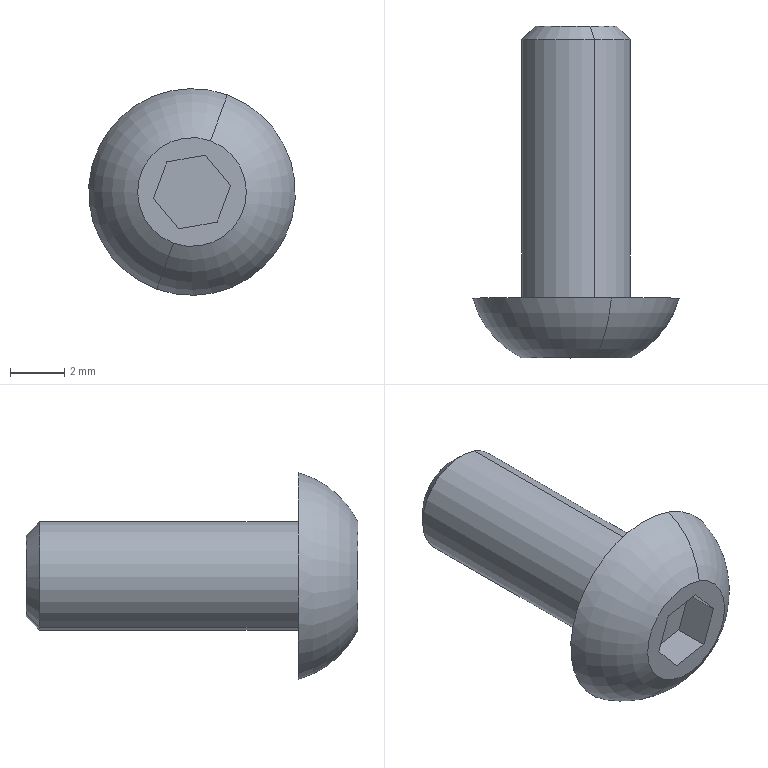Component | SolidWorks | SocketFlatHeadCapScrewM4_10-2 | 1 solid | 16 faces | box 7.6 x 12.2 x 7.6 mm | volume 188 mm3 | plane 10 | cone 2 | cylinder 2 | torus 2 | commonest cylinder face diameters 4 x2
STEP:
#1=CARTESIAN_POINT('',(-0.02018,0.5787,-2.238));
#2=VERTEX_POINT('',#1);
#3=CARTESIAN_POINT('',(0.02018,0.5787,-2.127));
#4=VERTEX_POINT('',#3);
#5=CARTESIAN_POINT('',(-0.,0.5787,-2.183));
#6=DIRECTION('',(0.,1.,0.));
#7=DIRECTION('',(-0.3417,0.,-0.9398));
#8=AXIS2_PLACEMENT_3D('',#5,#6,#7);
#9=CIRCLE('',#8,0.05906);
#10=EDGE_CURVE('',#2,#4,#9,.T.);
#11=ORIENTED_EDGE('',*,*,#10,.F.);
#12=CARTESIAN_POINT('',(-0.02691,0.5591,-2.257));
#13=VERTEX_POINT('',#12);
#14=CARTESIAN_POINT('',(-0.02018,0.5787,-2.238));
#15=DIRECTION('',(-0.2416,-0.7071,-0.6645));
#16=VECTOR('',#15,39.37);
#17=LINE('',#14,#16);
#18=EDGE_CURVE('',#2,#13,#17,.T.);
#19=ORIENTED_EDGE('',*,*,#18,.T.);
#20=CARTESIAN_POINT('',(0.02691,0.5591,-2.109));
#21=VERTEX_POINT('',#20);
#22=CARTESIAN_POINT('',(-0.,0.5591,-2.183));
#23=DIRECTION('',(-0.,-1.,-0.));
#24=DIRECTION('',(-0.3417,0.,-0.9398));
#25=AXIS2_PLACEMENT_3D('',#22,#23,#24);
#26=CIRCLE('',#25,0.07874);
#27=EDGE_CURVE('',#21,#13,#26,.T.);
#28=ORIENTED_EDGE('',*,*,#27,.F.);
#29=CARTESIAN_POINT('',(0.02018,0.5787,-2.127));
#30=DIRECTION('',(0.2416,-0.7071,0.6645));
#31=VECTOR('',#30,39.37);
#32=LINE('',#29,#31);
#33=EDGE_CURVE('',#4,#21,#32,.T.);
#34=ORIENTED_EDGE('',*,*,#33,.F.);
#35=EDGE_LOOP('',(#11,#19,#28,#34));
#36=FACE_OUTER_BOUND('',#35,.T.);
#37=CARTESIAN_POINT('',(-0.,0.5787,-2.183));
#38=DIRECTION('',(-0.,-1.,-0.));
#39=DIRECTION('',(0.3417,0.,0.9398));
#40=AXIS2_PLACEMENT_3D('',#37,#38,#39);
#41=CONICAL_SURFACE('',#40,0.05906,0.7854);
#42=ADVANCED_FACE('',(#36),#41,.T.);
#43=CARTESIAN_POINT('',(-0.02691,0.185,-2.257));
#44=VERTEX_POINT('',#43);
#45=CARTESIAN_POINT('',(0.02691,0.185,-2.109));
#46=VERTEX_POINT('',#45);
#47=CARTESIAN_POINT('',(-0.,0.185,-2.183));
#48=DIRECTION('',(0.,1.,0.));
#49=DIRECTION('',(-0.3417,0.,-0.9398));
#50=AXIS2_PLACEMENT_3D('',#47,#48,#49);
#51=CIRCLE('',#50,0.07874);
#52=EDGE_CURVE('',#44,#46,#51,.T.);
#53=ORIENTED_EDGE('',*,*,#52,.T.);
#54=CARTESIAN_POINT('',(0.02691,0.09843,-2.109));
#55=DIRECTION('',(0.,1.,0.));
#56=VECTOR('',#55,39.37);
#57=LINE('',#54,#56);
#58=EDGE_CURVE('',#46,#21,#57,.T.);
#59=ORIENTED_EDGE('',*,*,#58,.T.);
#60=ORIENTED_EDGE('',*,*,#27,.T.);
#61=CARTESIAN_POINT('',(-0.02691,0.09843,-2.257));
#62=DIRECTION('',(0.,1.,0.));
#63=VECTOR('',#62,39.37);
#64=LINE('',#61,#63);
#65=EDGE_CURVE('',#44,#13,#64,.T.);
#66=ORIENTED_EDGE('',*,*,#65,.F.);
#67=EDGE_LOOP('',(#53,#59,#60,#66));
#68=FACE_OUTER_BOUND('',#67,.T.);
#69=CARTESIAN_POINT('',(-0.,0.09843,-2.183));
#70=DIRECTION('',(0.,1.,0.));
#71=DIRECTION('',(-0.3417,0.,-0.9398));
#72=AXIS2_PLACEMENT_3D('',#69,#70,#71);
#73=CYLINDRICAL_SURFACE('',#72,0.07874);
#74=ADVANCED_FACE('',(#68),#73,.T.);
#75=CARTESIAN_POINT('',(-0.02691,0.09843,-2.257));
#76=VERTEX_POINT('',#75);
#77=CARTESIAN_POINT('',(0.02691,0.09843,-2.109));
#78=VERTEX_POINT('',#77);
#79=CARTESIAN_POINT('',(-0.,0.09843,-2.183));
#80=DIRECTION('',(0.,1.,0.));
#81=DIRECTION('',(-0.3417,0.,-0.9398));
#82=AXIS2_PLACEMENT_3D('',#79,#80,#81);
#83=CIRCLE('',#82,0.07874);
#84=EDGE_CURVE('',#76,#78,#83,.T.);
#85=ORIENTED_EDGE('',*,*,#84,.T.);
#86=CARTESIAN_POINT('',(0.05113,0.185,-2.042));
#87=VERTEX_POINT('',#86);
#88=CARTESIAN_POINT('',(0.005712,0.2215,-2.167));
#89=DIRECTION('',(-0.9398,0.,0.3417));
#90=DIRECTION('',(0.3417,0.,0.9398));
#91=AXIS2_PLACEMENT_3D('',#88,#89,#90);
#92=CIRCLE('',#91,0.1378);
#93=EDGE_CURVE('',#78,#87,#92,.T.);
#94=ORIENTED_EDGE('',*,*,#93,.T.);
#95=CARTESIAN_POINT('',(-0.05113,0.185,-2.324));
#96=VERTEX_POINT('',#95);
#97=CARTESIAN_POINT('',(-0.,0.185,-2.183));
#98=DIRECTION('',(0.,1.,0.));
#99=DIRECTION('',(-0.3417,0.,-0.9398));
#100=AXIS2_PLACEMENT_3D('',#97,#98,#99);
#101=CIRCLE('',#100,0.1496);
#102=EDGE_CURVE('',#96,#87,#101,.T.);
#103=ORIENTED_EDGE('',*,*,#102,.F.);
#104=CARTESIAN_POINT('',(-0.005712,0.2215,-2.199));
#105=DIRECTION('',(0.9398,-0.,-0.3417));
#106=DIRECTION('',(-0.3417,0.,-0.9398));
#107=AXIS2_PLACEMENT_3D('',#104,#105,#106);
#108=CIRCLE('',#107,0.1378);
#109=EDGE_CURVE('',#76,#96,#108,.T.);
#110=ORIENTED_EDGE('',*,*,#109,.F.);
#111=EDGE_LOOP('',(#85,#94,#103,#110));
#112=FACE_OUTER_BOUND('',#111,.T.);
#113=CARTESIAN_POINT('',(-0.,0.2215,-2.183));
#114=DIRECTION('',(0.,1.,0.));
#115=DIRECTION('',(-0.3417,0.,-0.9398));
#116=AXIS2_PLACEMENT_3D('',#113,#114,#115);
#117=TOROIDAL_SURFACE('',#116,0.01671,0.1378);
#118=ADVANCED_FACE('',(#112),#117,.T.);
#119=CARTESIAN_POINT('',(0.05596,0.09843,-2.173));
#120=VERTEX_POINT('',#119);
#121=CARTESIAN_POINT('',(0.01942,0.09843,-2.13));
#122=VERTEX_POINT('',#121);
#123=CARTESIAN_POINT('',(0.05596,0.09843,-2.173));
#124=DIRECTION('',(-0.643,0.,0.7658));
#125=VECTOR('',#124,39.37);
#126=LINE('',#123,#125);
#127=EDGE_CURVE('',#120,#122,#126,.T.);
#128=ORIENTED_EDGE('',*,*,#127,.F.);
#129=CARTESIAN_POINT('',(0.03654,0.09843,-2.226));
#130=VERTEX_POINT('',#129);
#131=CARTESIAN_POINT('',(0.03654,0.09843,-2.226));
#132=DIRECTION('',(0.3417,-0.,0.9398));
#133=VECTOR('',#132,39.37);
#134=LINE('',#131,#133);
#135=EDGE_CURVE('',#130,#120,#134,.T.);
#136=ORIENTED_EDGE('',*,*,#135,.F.);
#137=CARTESIAN_POINT('',(-0.01942,0.09843,-2.236));
#138=VERTEX_POINT('',#137);
#139=CARTESIAN_POINT('',(-0.01942,0.09843,-2.236));
#140=DIRECTION('',(0.9848,-0.,0.174));
#141=VECTOR('',#140,39.37);
#142=LINE('',#139,#141);
#143=EDGE_CURVE('',#138,#130,#142,.T.);
#144=ORIENTED_EDGE('',*,*,#143,.F.);
#145=CARTESIAN_POINT('',(-0.05596,0.09843,-2.193));
#146=VERTEX_POINT('',#145);
#147=CARTESIAN_POINT('',(-0.05596,0.09843,-2.193));
#148=DIRECTION('',(0.643,-0.,-0.7658));
#149=VECTOR('',#148,39.37);
#150=LINE('',#147,#149);
#151=EDGE_CURVE('',#146,#138,#150,.T.);
#152=ORIENTED_EDGE('',*,*,#151,.F.);
#153=CARTESIAN_POINT('',(-0.03654,0.09843,-2.139));
#154=VERTEX_POINT('',#153);
#155=CARTESIAN_POINT('',(-0.03654,0.09843,-2.139));
#156=DIRECTION('',(-0.3417,0.,-0.9398));
#157=VECTOR('',#156,39.37);
#158=LINE('',#155,#157);
#159=EDGE_CURVE('',#154,#146,#158,.T.);
#160=ORIENTED_EDGE('',*,*,#159,.F.);
#161=CARTESIAN_POINT('',(0.01942,0.09843,-2.13));
#162=DIRECTION('',(-0.9848,0.,-0.174));
#163=VECTOR('',#162,39.37);
#164=LINE('',#161,#163);
#165=EDGE_CURVE('',#122,#154,#164,.T.);
#166=ORIENTED_EDGE('',*,*,#165,.F.);
#167=EDGE_LOOP('',(#128,#136,#144,#152,#160,#166));
#168=FACE_BOUND('',#167,.T.);
#169=ORIENTED_EDGE('',*,*,#84,.F.);
#170=CARTESIAN_POINT('',(-0.,0.09843,-2.183));
#171=DIRECTION('',(0.,1.,0.));
#172=DIRECTION('',(-0.3417,0.,-0.9398));
#173=AXIS2_PLACEMENT_3D('',#170,#171,#172);
#174=CIRCLE('',#173,0.07874);
#175=EDGE_CURVE('',#78,#76,#174,.T.);
#176=ORIENTED_EDGE('',*,*,#175,.F.);
#177=EDGE_LOOP('',(#169,#176));
#178=FACE_OUTER_BOUND('',#177,.T.);
#179=CARTESIAN_POINT('',(-0.,0.09843,-2.183));
#180=DIRECTION('',(-0.,-1.,-0.));
#181=DIRECTION('',(0.3417,-0.,0.9398));
#182=AXIS2_PLACEMENT_3D('',#179,#180,#181);
#183=PLANE('',#182);
#184=ADVANCED_FACE('',(#168,#178),#183,.T.);
#185=ORIENTED_EDGE('',*,*,#93,.F.);
#186=ORIENTED_EDGE('',*,*,#175,.T.);
#187=ORIENTED_EDGE('',*,*,#109,.T.);
#188=CARTESIAN_POINT('',(-0.,0.185,-2.183));
#189=DIRECTION('',(0.,1.,0.));
#190=DIRECTION('',(-0.3417,0.,-0.9398));
#191=AXIS2_PLACEMENT_3D('',#188,#189,#190);
#192=CIRCLE('',#191,0.1496);
#193=EDGE_CURVE('',#87,#96,#192,.T.);
#194=ORIENTED_EDGE('',*,*,#193,.F.);
#195=EDGE_LOOP('',(#185,#186,#187,#194));
#196=FACE_OUTER_BOUND('',#195,.T.);
#197=CARTESIAN_POINT('',(-0.,0.2215,-2.183));
#198=DIRECTION('',(0.,1.,0.));
#199=DIRECTION('',(-0.3417,0.,-0.9398));
#200=AXIS2_PLACEMENT_3D('',#197,#198,#199);
#201=TOROIDAL_SURFACE('',#200,0.01671,0.1378);
#202=ADVANCED_FACE('',(#196),#201,.T.);
#203=ORIENTED_EDGE('',*,*,#102,.T.);
#204=ORIENTED_EDGE('',*,*,#193,.T.);
#205=EDGE_LOOP('',(#203,#204));
#206=FACE_OUTER_BOUND('',#205,.T.);
#207=ORIENTED_EDGE('',*,*,#52,.F.);
#208=CARTESIAN_POINT('',(-0.,0.185,-2.183));
#209=DIRECTION('',(0.,1.,0.));
#210=DIRECTION('',(-0.3417,0.,-0.9398));
#211=AXIS2_PLACEMENT_3D('',#208,#209,#210);
#212=CIRCLE('',#211,0.07874);
#213=EDGE_CURVE('',#46,#44,#212,.T.);
#214=ORIENTED_EDGE('',*,*,#213,.F.);
#215=EDGE_LOOP('',(#207,#214));
#216=FACE_BOUND('',#215,.T.);
#217=CARTESIAN_POINT('',(-0.1406,0.185,-2.132));
#218=DIRECTION('',(0.,1.,0.));
#219=DIRECTION('',(-0.3417,0.,-0.9398));
#220=AXIS2_PLACEMENT_3D('',#217,#218,#219);
#221=PLANE('',#220);
#222=ADVANCED_FACE('',(#206,#216),#221,.T.);
#223=ORIENTED_EDGE('',*,*,#58,.F.);
#224=ORIENTED_EDGE('',*,*,#213,.T.);
#225=ORIENTED_EDGE('',*,*,#65,.T.);
#226=CARTESIAN_POINT('',(-0.,0.5591,-2.183));
#227=DIRECTION('',(-0.,-1.,-0.));
#228=DIRECTION('',(-0.3417,0.,-0.9398));
#229=AXIS2_PLACEMENT_3D('',#226,#227,#228);
#230=CIRCLE('',#229,0.07874);
#231=EDGE_CURVE('',#13,#21,#230,.T.);
#232=ORIENTED_EDGE('',*,*,#231,.T.);
#233=EDGE_LOOP('',(#223,#224,#225,#232));
#234=FACE_OUTER_BOUND('',#233,.T.);
#235=CARTESIAN_POINT('',(-0.,0.09843,-2.183));
#236=DIRECTION('',(0.,1.,0.));
#237=DIRECTION('',(-0.3417,0.,-0.9398));
#238=AXIS2_PLACEMENT_3D('',#235,#236,#237);
#239=CYLINDRICAL_SURFACE('',#238,0.07874);
#240=ADVANCED_FACE('',(#234),#239,.T.);
#241=CARTESIAN_POINT('',(-0.,0.5787,-2.183));
#242=DIRECTION('',(0.,1.,0.));
#243=DIRECTION('',(-0.3417,0.,-0.9398));
#244=AXIS2_PLACEMENT_3D('',#241,#242,#243);
#245=CIRCLE('',#244,0.05906);
#246=EDGE_CURVE('',#4,#2,#245,.T.);
#247=ORIENTED_EDGE('',*,*,#246,.T.);
#248=ORIENTED_EDGE('',*,*,#10,.T.);
#249=EDGE_LOOP('',(#247,#248));
#250=FACE_OUTER_BOUND('',#249,.T.);
#251=CARTESIAN_POINT('',(-0.074,0.5787,-2.156));
#252=DIRECTION('',(0.,1.,0.));
#253=DIRECTION('',(-0.3417,0.,-0.9398));
#254=AXIS2_PLACEMENT_3D('',#251,#252,#253);
#255=PLANE('',#254);
#256=ADVANCED_FACE('',(#250),#255,.T.);
#257=ORIENTED_EDGE('',*,*,#127,.T.);
#258=CARTESIAN_POINT('',(0.01942,0.1496,-2.13));
#259=VERTEX_POINT('',#258);
#260=CARTESIAN_POINT('',(0.01942,0.1496,-2.13));
#261=DIRECTION('',(-0.,-1.,-0.));
#262=VECTOR('',#261,39.37);
#263=LINE('',#260,#262);
#264=EDGE_CURVE('',#259,#122,#263,.T.);
#265=ORIENTED_EDGE('',*,*,#264,.F.);
#266=CARTESIAN_POINT('',(0.05596,0.1496,-2.173));
#267=VERTEX_POINT('',#266);
#268=CARTESIAN_POINT('',(0.05596,0.1496,-2.173));
#269=DIRECTION('',(-0.643,0.,0.7658));
#270=VECTOR('',#269,39.37);
#271=LINE('',#268,#270);
#272=EDGE_CURVE('',#267,#259,#271,.T.);
#273=ORIENTED_EDGE('',*,*,#272,.F.);
#274=CARTESIAN_POINT('',(0.05596,0.1496,-2.173));
#275=DIRECTION('',(-0.,-1.,-0.));
#276=VECTOR('',#275,39.37);
#277=LINE('',#274,#276);
#278=EDGE_CURVE('',#267,#120,#277,.T.);
#279=ORIENTED_EDGE('',*,*,#278,.T.);
#280=EDGE_LOOP('',(#257,#265,#273,#279));
#281=FACE_OUTER_BOUND('',#280,.T.);
#282=CARTESIAN_POINT('',(0.05596,0.1496,-2.173));
#283=DIRECTION('',(0.7658,-0.,0.643));
#284=DIRECTION('',(0.643,-0.,-0.7658));
#285=AXIS2_PLACEMENT_3D('',#282,#283,#284);
#286=PLANE('',#285);
#287=ADVANCED_FACE('',(#281),#286,.F.);
#288=ORIENTED_EDGE('',*,*,#135,.T.);
#289=ORIENTED_EDGE('',*,*,#278,.F.);
#290=CARTESIAN_POINT('',(0.03654,0.1496,-2.226));
#291=VERTEX_POINT('',#290);
#292=CARTESIAN_POINT('',(0.03654,0.1496,-2.226));
#293=DIRECTION('',(0.3417,-0.,0.9398));
#294=VECTOR('',#293,39.37);
#295=LINE('',#292,#294);
#296=EDGE_CURVE('',#291,#267,#295,.T.);
#297=ORIENTED_EDGE('',*,*,#296,.F.);
#298=CARTESIAN_POINT('',(0.03654,0.1496,-2.226));
#299=DIRECTION('',(-0.,-1.,-0.));
#300=VECTOR('',#299,39.37);
#301=LINE('',#298,#300);
#302=EDGE_CURVE('',#291,#130,#301,.T.);
#303=ORIENTED_EDGE('',*,*,#302,.T.);
#304=EDGE_LOOP('',(#288,#289,#297,#303));
#305=FACE_OUTER_BOUND('',#304,.T.);
#306=CARTESIAN_POINT('',(0.03654,0.1496,-2.226));
#307=DIRECTION('',(0.9398,-0.,-0.3417));
#308=DIRECTION('',(-0.3417,0.,-0.9398));
#309=AXIS2_PLACEMENT_3D('',#306,#307,#308);
#310=PLANE('',#309);
#311=ADVANCED_FACE('',(#305),#310,.F.);
#312=ORIENTED_EDGE('',*,*,#143,.T.);
#313=ORIENTED_EDGE('',*,*,#302,.F.);
#314=CARTESIAN_POINT('',(-0.01942,0.1496,-2.236));
#315=VERTEX_POINT('',#314);
#316=CARTESIAN_POINT('',(-0.01942,0.1496,-2.236));
#317=DIRECTION('',(0.9848,-0.,0.174));
#318=VECTOR('',#317,39.37);
#319=LINE('',#316,#318);
#320=EDGE_CURVE('',#315,#291,#319,.T.);
#321=ORIENTED_EDGE('',*,*,#320,.F.);
#322=CARTESIAN_POINT('',(-0.01942,0.1496,-2.236));
#323=DIRECTION('',(-0.,-1.,-0.));
#324=VECTOR('',#323,39.37);
#325=LINE('',#322,#324);
#326=EDGE_CURVE('',#315,#138,#325,.T.);
#327=ORIENTED_EDGE('',*,*,#326,.T.);
#328=EDGE_LOOP('',(#312,#313,#321,#327));
#329=FACE_OUTER_BOUND('',#328,.T.);
#330=CARTESIAN_POINT('',(-0.01942,0.1496,-2.236));
#331=DIRECTION('',(0.174,0.,-0.9848));
#332=DIRECTION('',(-0.9848,0.,-0.174));
#333=AXIS2_PLACEMENT_3D('',#330,#331,#332);
#334=PLANE('',#333);
#335=ADVANCED_FACE('',(#329),#334,.F.);
#336=ORIENTED_EDGE('',*,*,#151,.T.);
#337=ORIENTED_EDGE('',*,*,#326,.F.);
#338=CARTESIAN_POINT('',(-0.05596,0.1496,-2.193));
#339=VERTEX_POINT('',#338);
#340=CARTESIAN_POINT('',(-0.05596,0.1496,-2.193));
#341=DIRECTION('',(0.643,-0.,-0.7658));
#342=VECTOR('',#341,39.37);
#343=LINE('',#340,#342);
#344=EDGE_CURVE('',#339,#315,#343,.T.);
#345=ORIENTED_EDGE('',*,*,#344,.F.);
#346=CARTESIAN_POINT('',(-0.05596,0.1496,-2.193));
#347=DIRECTION('',(-0.,-1.,-0.));
#348=VECTOR('',#347,39.37);
#349=LINE('',#346,#348);
#350=EDGE_CURVE('',#339,#146,#349,.T.);
#351=ORIENTED_EDGE('',*,*,#350,.T.);
#352=EDGE_LOOP('',(#336,#337,#345,#351));
#353=FACE_OUTER_BOUND('',#352,.T.);
#354=CARTESIAN_POINT('',(-0.05596,0.1496,-2.193));
#355=DIRECTION('',(-0.7658,0.,-0.643));
#356=DIRECTION('',(-0.643,0.,0.7658));
#357=AXIS2_PLACEMENT_3D('',#354,#355,#356);
#358=PLANE('',#357);
#359=ADVANCED_FACE('',(#353),#358,.F.);
#360=ORIENTED_EDGE('',*,*,#159,.T.);
#361=ORIENTED_EDGE('',*,*,#350,.F.);
#362=CARTESIAN_POINT('',(-0.03654,0.1496,-2.139));
#363=VERTEX_POINT('',#362);
#364=CARTESIAN_POINT('',(-0.03654,0.1496,-2.139));
#365=DIRECTION('',(-0.3417,0.,-0.9398));
#366=VECTOR('',#365,39.37);
#367=LINE('',#364,#366);
#368=EDGE_CURVE('',#363,#339,#367,.T.);
#369=ORIENTED_EDGE('',*,*,#368,.F.);
#370=CARTESIAN_POINT('',(-0.03654,0.1496,-2.139));
#371=DIRECTION('',(-0.,-1.,-0.));
#372=VECTOR('',#371,39.37);
#373=LINE('',#370,#372);
#374=EDGE_CURVE('',#363,#154,#373,.T.);
#375=ORIENTED_EDGE('',*,*,#374,.T.);
#376=EDGE_LOOP('',(#360,#361,#369,#375));
#377=FACE_OUTER_BOUND('',#376,.T.);
#378=CARTESIAN_POINT('',(-0.03654,0.1496,-2.139));
#379=DIRECTION('',(-0.9398,0.,0.3417));
#380=DIRECTION('',(0.3417,-0.,0.9398));
#381=AXIS2_PLACEMENT_3D('',#378,#379,#380);
#382=PLANE('',#381);
#383=ADVANCED_FACE('',(#377),#382,.F.);
#384=ORIENTED_EDGE('',*,*,#165,.T.);
#385=ORIENTED_EDGE('',*,*,#374,.F.);
#386=CARTESIAN_POINT('',(0.01942,0.1496,-2.13));
#387=DIRECTION('',(-0.9848,0.,-0.174));
#388=VECTOR('',#387,39.37);
#389=LINE('',#386,#388);
#390=EDGE_CURVE('',#259,#363,#389,.T.);
#391=ORIENTED_EDGE('',*,*,#390,.F.);
#392=ORIENTED_EDGE('',*,*,#264,.T.);
#393=EDGE_LOOP('',(#384,#385,#391,#392));
#394=FACE_OUTER_BOUND('',#393,.T.);
#395=CARTESIAN_POINT('',(0.01942,0.1496,-2.13));
#396=DIRECTION('',(-0.174,-0.,0.9848));
#397=DIRECTION('',(0.9848,-0.,0.174));
#398=AXIS2_PLACEMENT_3D('',#395,#396,#397);
#399=PLANE('',#398);
#400=ADVANCED_FACE('',(#394),#399,.F.);
#401=ORIENTED_EDGE('',*,*,#272,.T.);
#402=ORIENTED_EDGE('',*,*,#390,.T.);
#403=ORIENTED_EDGE('',*,*,#368,.T.);
#404=ORIENTED_EDGE('',*,*,#344,.T.);
#405=ORIENTED_EDGE('',*,*,#320,.T.);
#406=ORIENTED_EDGE('',*,*,#296,.T.);
#407=EDGE_LOOP('',(#401,#402,#403,#404,#405,#406));
#408=FACE_OUTER_BOUND('',#407,.T.);
#409=CARTESIAN_POINT('',(-0.01712,0.1496,-2.086));
#410=DIRECTION('',(-0.,-1.,-0.));
#411=DIRECTION('',(0.3417,-0.,0.9398));
#412=AXIS2_PLACEMENT_3D('',#409,#410,#411);
#413=PLANE('',#412);
#414=ADVANCED_FACE('',(#408),#413,.T.);
#415=ORIENTED_EDGE('',*,*,#18,.F.);
#416=ORIENTED_EDGE('',*,*,#246,.F.);
#417=ORIENTED_EDGE('',*,*,#33,.T.);
#418=ORIENTED_EDGE('',*,*,#231,.F.);
#419=EDGE_LOOP('',(#415,#416,#417,#418));
#420=FACE_OUTER_BOUND('',#419,.T.);
#421=CARTESIAN_POINT('',(-0.,0.5787,-2.183));
#422=DIRECTION('',(-0.,-1.,-0.));
#423=DIRECTION('',(0.3417,0.,0.9398));
#424=AXIS2_PLACEMENT_3D('',#421,#422,#423);
#425=CONICAL_SURFACE('',#424,0.05906,0.7854);
#426=ADVANCED_FACE('',(#420),#425,.T.);
#427=CLOSED_SHELL('',(#42,#74,#118,#184,#202,#222,#240,#256,#287,#311,#335,#359,#383,#400,#414,#426));
#428=MANIFOLD_SOLID_BREP('',#427);
#429=CARTESIAN_POINT('',(0.,0.,0.));
#430=DIRECTION('',(0.,0.,1.));
#431=DIRECTION('',(1.,0.,0.));
#432=AXIS2_PLACEMENT_3D('',#429,#430,#431);
#433=(LENGTH_UNIT()NAMED_UNIT(*)SI_UNIT($,.METRE.));
#434=LENGTH_MEASURE_WITH_UNIT(LENGTH_MEASURE(0.0254),#433);
#435=DIMENSIONAL_EXPONENTS(1.,0.,0.,0.,0.,0.,0.);
#436=(CONVERSION_BASED_UNIT('',#434)LENGTH_UNIT()NAMED_UNIT(#435));
#437=UNCERTAINTY_MEASURE_WITH_UNIT(LENGTH_MEASURE(0.00001),#436,'','');
#438=(NAMED_UNIT(*)PLANE_ANGLE_UNIT()SI_UNIT($,.RADIAN.));
#439=(NAMED_UNIT(*)SI_UNIT($,.STERADIAN.)SOLID_ANGLE_UNIT());
#440=(GEOMETRIC_REPRESENTATION_CONTEXT(3)GLOBAL_UNCERTAINTY_ASSIGNED_CONTEXT((#437))GLOBAL_UNIT_ASSIGNED_CONTEXT((#436,#438,#439))REPRESENTATION_CONTEXT('',''));
#441=ADVANCED_BREP_SHAPE_REPRESENTATION('',(#428,#432),#440);
#442=COLOUR_RGB('',0.7922,0.8196,0.9333);
#443=FILL_AREA_STYLE_COLOUR('',#442);
#444=FILL_AREA_STYLE('',(#443));
#445=SURFACE_STYLE_FILL_AREA(#444);
#446=SURFACE_SIDE_STYLE('',(#445));
#447=SURFACE_STYLE_USAGE(.BOTH.,#446);
#448=PRESENTATION_STYLE_ASSIGNMENT((#447));
#449=STYLED_ITEM('',(#448),#428);
#450=PRESENTATION_LAYER_ASSIGNMENT('','',(#449));
#451=(LENGTH_UNIT()NAMED_UNIT(*)SI_UNIT($,.METRE.));
#452=LENGTH_MEASURE_WITH_UNIT(LENGTH_MEASURE(0.0254),#451);
#453=DIMENSIONAL_EXPONENTS(1.,0.,0.,0.,0.,0.,0.);
#454=(CONVERSION_BASED_UNIT('',#452)LENGTH_UNIT()NAMED_UNIT(#453));
#455=UNCERTAINTY_MEASURE_WITH_UNIT(LENGTH_MEASURE(0.00001),#454,'','');
#456=(NAMED_UNIT(*)PLANE_ANGLE_UNIT()SI_UNIT($,.RADIAN.));
#457=(NAMED_UNIT(*)SI_UNIT($,.STERADIAN.)SOLID_ANGLE_UNIT());
#458=(GEOMETRIC_REPRESENTATION_CONTEXT(3)GLOBAL_UNCERTAINTY_ASSIGNED_CONTEXT((#455))GLOBAL_UNIT_ASSIGNED_CONTEXT((#454,#456,#457))REPRESENTATION_CONTEXT('',''));
#459=MECHANICAL_DESIGN_GEOMETRIC_PRESENTATION_REPRESENTATION('',(#449),#458);